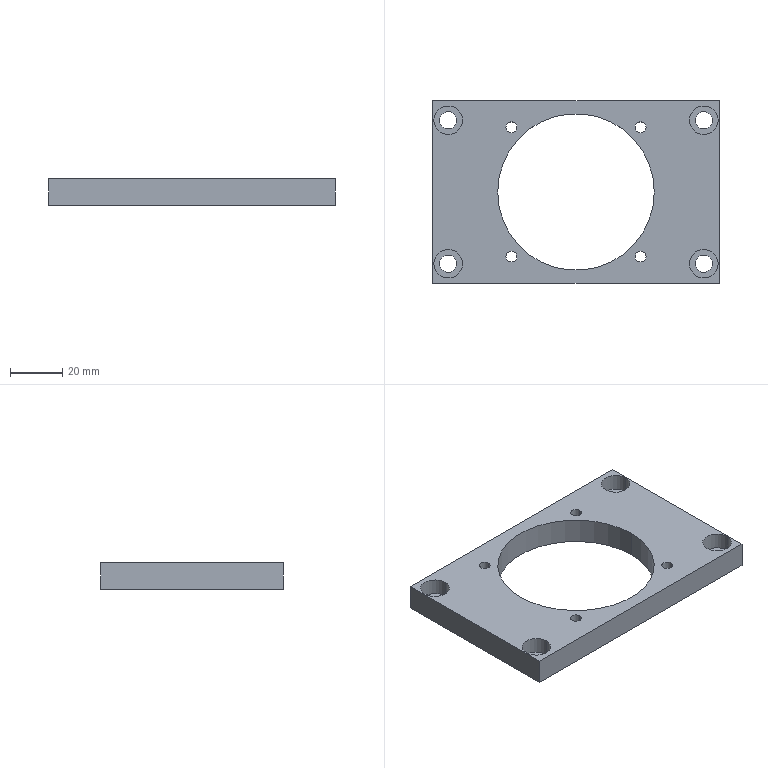Component | SolidWorks | ServoDriveMotorModule-1_WT-FLD-EJG-1212-00-019-1 | 1 solid | 36 faces | box 110 x 70 x 10 mm | volume 45246 mm3 | cylinder 26 | plane 10 | commonest cylinder face diameters 11 x8 6.6 x8 4.2 x8 60 x2 | material AISI 1045 Steel, cold drawn
STEP:
#1=COLOUR_RGB('',0.7922,0.8196,0.9333);
#2=FILL_AREA_STYLE_COLOUR('',#1);
#3=FILL_AREA_STYLE('',(#2));
#4=SURFACE_STYLE_FILL_AREA(#3);
#5=SURFACE_SIDE_STYLE('',(#4));
#6=SURFACE_STYLE_USAGE(.BOTH.,#5);
#7=PRESENTATION_STYLE_ASSIGNMENT((#6));
#8=CARTESIAN_POINT('',(-2.146,1.083,5.26));
#9=VERTEX_POINT('',#8);
#10=CARTESIAN_POINT('',(-1.713,1.083,5.26));
#11=VERTEX_POINT('',#10);
#12=CARTESIAN_POINT('',(-1.929,1.083,5.26));
#13=DIRECTION('',(0.,0.,1.));
#14=DIRECTION('',(1.,0.,0.));
#15=AXIS2_PLACEMENT_3D('',#12,#13,#14);
#16=CIRCLE('',#15,0.2165);
#17=EDGE_CURVE('',#9,#11,#16,.T.);
#18=ORIENTED_EDGE('',*,*,#17,.F.);
#19=CARTESIAN_POINT('',(-2.146,1.083,5.512));
#20=VERTEX_POINT('',#19);
#21=CARTESIAN_POINT('',(-2.146,1.083,5.512));
#22=DIRECTION('',(0.,0.,1.));
#23=VECTOR('',#22,39.37);
#24=LINE('',#21,#23);
#25=EDGE_CURVE('',#9,#20,#24,.T.);
#26=ORIENTED_EDGE('',*,*,#25,.T.);
#27=CARTESIAN_POINT('',(-1.713,1.083,5.512));
#28=VERTEX_POINT('',#27);
#29=CARTESIAN_POINT('',(-1.929,1.083,5.512));
#30=DIRECTION('',(0.,0.,1.));
#31=DIRECTION('',(1.,0.,0.));
#32=AXIS2_PLACEMENT_3D('',#29,#30,#31);
#33=CIRCLE('',#32,0.2165);
#34=EDGE_CURVE('',#20,#28,#33,.T.);
#35=ORIENTED_EDGE('',*,*,#34,.T.);
#36=CARTESIAN_POINT('',(-1.713,1.083,5.512));
#37=DIRECTION('',(0.,0.,1.));
#38=VECTOR('',#37,39.37);
#39=LINE('',#36,#38);
#40=EDGE_CURVE('',#11,#28,#39,.T.);
#41=ORIENTED_EDGE('',*,*,#40,.F.);
#42=EDGE_LOOP('',(#18,#26,#35,#41));
#43=FACE_OUTER_BOUND('',#42,.T.);
#44=CARTESIAN_POINT('',(-1.929,1.083,5.512));
#45=DIRECTION('',(0.,0.,1.));
#46=DIRECTION('',(1.,0.,0.));
#47=AXIS2_PLACEMENT_3D('',#44,#45,#46);
#48=CYLINDRICAL_SURFACE('',#47,0.2165);
#49=ADVANCED_FACE('',(#43),#48,.F.);
#50=CARTESIAN_POINT('',(-2.059,1.083,5.118));
#51=VERTEX_POINT('',#50);
#52=CARTESIAN_POINT('',(-1.799,1.083,5.118));
#53=VERTEX_POINT('',#52);
#54=CARTESIAN_POINT('',(-1.929,1.083,5.118));
#55=DIRECTION('',(0.,0.,1.));
#56=DIRECTION('',(1.,0.,0.));
#57=AXIS2_PLACEMENT_3D('',#54,#55,#56);
#58=CIRCLE('',#57,0.1299);
#59=EDGE_CURVE('',#51,#53,#58,.T.);
#60=ORIENTED_EDGE('',*,*,#59,.F.);
#61=CARTESIAN_POINT('',(-2.059,1.083,5.26));
#62=VERTEX_POINT('',#61);
#63=CARTESIAN_POINT('',(-2.059,1.083,5.512));
#64=DIRECTION('',(0.,0.,1.));
#65=VECTOR('',#64,39.37);
#66=LINE('',#63,#65);
#67=EDGE_CURVE('',#51,#62,#66,.T.);
#68=ORIENTED_EDGE('',*,*,#67,.T.);
#69=CARTESIAN_POINT('',(-1.799,1.083,5.26));
#70=VERTEX_POINT('',#69);
#71=CARTESIAN_POINT('',(-1.929,1.083,5.26));
#72=DIRECTION('',(0.,0.,1.));
#73=DIRECTION('',(1.,0.,0.));
#74=AXIS2_PLACEMENT_3D('',#71,#72,#73);
#75=CIRCLE('',#74,0.1299);
#76=EDGE_CURVE('',#62,#70,#75,.T.);
#77=ORIENTED_EDGE('',*,*,#76,.T.);
#78=CARTESIAN_POINT('',(-1.799,1.083,5.512));
#79=DIRECTION('',(0.,0.,1.));
#80=VECTOR('',#79,39.37);
#81=LINE('',#78,#80);
#82=EDGE_CURVE('',#53,#70,#81,.T.);
#83=ORIENTED_EDGE('',*,*,#82,.F.);
#84=EDGE_LOOP('',(#60,#68,#77,#83));
#85=FACE_OUTER_BOUND('',#84,.T.);
#86=CARTESIAN_POINT('',(-1.929,1.083,5.512));
#87=DIRECTION('',(0.,0.,1.));
#88=DIRECTION('',(1.,0.,0.));
#89=AXIS2_PLACEMENT_3D('',#86,#87,#88);
#90=CYLINDRICAL_SURFACE('',#89,0.1299);
#91=ADVANCED_FACE('',(#85),#90,.F.);
#92=CARTESIAN_POINT('',(-2.146,-1.083,5.26));
#93=VERTEX_POINT('',#92);
#94=CARTESIAN_POINT('',(-1.713,-1.083,5.26));
#95=VERTEX_POINT('',#94);
#96=CARTESIAN_POINT('',(-1.929,-1.083,5.26));
#97=DIRECTION('',(0.,0.,1.));
#98=DIRECTION('',(1.,0.,0.));
#99=AXIS2_PLACEMENT_3D('',#96,#97,#98);
#100=CIRCLE('',#99,0.2165);
#101=EDGE_CURVE('',#93,#95,#100,.T.);
#102=ORIENTED_EDGE('',*,*,#101,.F.);
#103=CARTESIAN_POINT('',(-2.146,-1.083,5.512));
#104=VERTEX_POINT('',#103);
#105=CARTESIAN_POINT('',(-2.146,-1.083,5.512));
#106=DIRECTION('',(0.,0.,1.));
#107=VECTOR('',#106,39.37);
#108=LINE('',#105,#107);
#109=EDGE_CURVE('',#93,#104,#108,.T.);
#110=ORIENTED_EDGE('',*,*,#109,.T.);
#111=CARTESIAN_POINT('',(-1.713,-1.083,5.512));
#112=VERTEX_POINT('',#111);
#113=CARTESIAN_POINT('',(-1.929,-1.083,5.512));
#114=DIRECTION('',(0.,0.,1.));
#115=DIRECTION('',(1.,0.,0.));
#116=AXIS2_PLACEMENT_3D('',#113,#114,#115);
#117=CIRCLE('',#116,0.2165);
#118=EDGE_CURVE('',#104,#112,#117,.T.);
#119=ORIENTED_EDGE('',*,*,#118,.T.);
#120=CARTESIAN_POINT('',(-1.713,-1.083,5.512));
#121=DIRECTION('',(0.,0.,1.));
#122=VECTOR('',#121,39.37);
#123=LINE('',#120,#122);
#124=EDGE_CURVE('',#95,#112,#123,.T.);
#125=ORIENTED_EDGE('',*,*,#124,.F.);
#126=EDGE_LOOP('',(#102,#110,#119,#125));
#127=FACE_OUTER_BOUND('',#126,.T.);
#128=CARTESIAN_POINT('',(-1.929,-1.083,5.512));
#129=DIRECTION('',(0.,0.,1.));
#130=DIRECTION('',(1.,0.,0.));
#131=AXIS2_PLACEMENT_3D('',#128,#129,#130);
#132=CYLINDRICAL_SURFACE('',#131,0.2165);
#133=ADVANCED_FACE('',(#127),#132,.F.);
#134=CARTESIAN_POINT('',(-2.059,-1.083,5.118));
#135=VERTEX_POINT('',#134);
#136=CARTESIAN_POINT('',(-1.799,-1.083,5.118));
#137=VERTEX_POINT('',#136);
#138=CARTESIAN_POINT('',(-1.929,-1.083,5.118));
#139=DIRECTION('',(0.,0.,1.));
#140=DIRECTION('',(1.,0.,0.));
#141=AXIS2_PLACEMENT_3D('',#138,#139,#140);
#142=CIRCLE('',#141,0.1299);
#143=EDGE_CURVE('',#135,#137,#142,.T.);
#144=ORIENTED_EDGE('',*,*,#143,.F.);
#145=CARTESIAN_POINT('',(-2.059,-1.083,5.26));
#146=VERTEX_POINT('',#145);
#147=CARTESIAN_POINT('',(-2.059,-1.083,5.512));
#148=DIRECTION('',(0.,0.,1.));
#149=VECTOR('',#148,39.37);
#150=LINE('',#147,#149);
#151=EDGE_CURVE('',#135,#146,#150,.T.);
#152=ORIENTED_EDGE('',*,*,#151,.T.);
#153=CARTESIAN_POINT('',(-1.799,-1.083,5.26));
#154=VERTEX_POINT('',#153);
#155=CARTESIAN_POINT('',(-1.929,-1.083,5.26));
#156=DIRECTION('',(0.,0.,1.));
#157=DIRECTION('',(1.,0.,0.));
#158=AXIS2_PLACEMENT_3D('',#155,#156,#157);
#159=CIRCLE('',#158,0.1299);
#160=EDGE_CURVE('',#146,#154,#159,.T.);
#161=ORIENTED_EDGE('',*,*,#160,.T.);
#162=CARTESIAN_POINT('',(-1.799,-1.083,5.512));
#163=DIRECTION('',(0.,0.,1.));
#164=VECTOR('',#163,39.37);
#165=LINE('',#162,#164);
#166=EDGE_CURVE('',#137,#154,#165,.T.);
#167=ORIENTED_EDGE('',*,*,#166,.F.);
#168=EDGE_LOOP('',(#144,#152,#161,#167));
#169=FACE_OUTER_BOUND('',#168,.T.);
#170=CARTESIAN_POINT('',(-1.929,-1.083,5.512));
#171=DIRECTION('',(0.,0.,1.));
#172=DIRECTION('',(1.,0.,0.));
#173=AXIS2_PLACEMENT_3D('',#170,#171,#172);
#174=CYLINDRICAL_SURFACE('',#173,0.1299);
#175=ADVANCED_FACE('',(#169),#174,.F.);
#176=CARTESIAN_POINT('',(1.713,-1.083,5.26));
#177=VERTEX_POINT('',#176);
#178=CARTESIAN_POINT('',(2.146,-1.083,5.26));
#179=VERTEX_POINT('',#178);
#180=CARTESIAN_POINT('',(1.929,-1.083,5.26));
#181=DIRECTION('',(0.,0.,1.));
#182=DIRECTION('',(1.,0.,0.));
#183=AXIS2_PLACEMENT_3D('',#180,#181,#182);
#184=CIRCLE('',#183,0.2165);
#185=EDGE_CURVE('',#177,#179,#184,.T.);
#186=ORIENTED_EDGE('',*,*,#185,.F.);
#187=CARTESIAN_POINT('',(1.713,-1.083,5.512));
#188=VERTEX_POINT('',#187);
#189=CARTESIAN_POINT('',(1.713,-1.083,5.512));
#190=DIRECTION('',(0.,0.,1.));
#191=VECTOR('',#190,39.37);
#192=LINE('',#189,#191);
#193=EDGE_CURVE('',#177,#188,#192,.T.);
#194=ORIENTED_EDGE('',*,*,#193,.T.);
#195=CARTESIAN_POINT('',(2.146,-1.083,5.512));
#196=VERTEX_POINT('',#195);
#197=CARTESIAN_POINT('',(1.929,-1.083,5.512));
#198=DIRECTION('',(0.,0.,1.));
#199=DIRECTION('',(1.,0.,0.));
#200=AXIS2_PLACEMENT_3D('',#197,#198,#199);
#201=CIRCLE('',#200,0.2165);
#202=EDGE_CURVE('',#188,#196,#201,.T.);
#203=ORIENTED_EDGE('',*,*,#202,.T.);
#204=CARTESIAN_POINT('',(2.146,-1.083,5.512));
#205=DIRECTION('',(0.,0.,1.));
#206=VECTOR('',#205,39.37);
#207=LINE('',#204,#206);
#208=EDGE_CURVE('',#179,#196,#207,.T.);
#209=ORIENTED_EDGE('',*,*,#208,.F.);
#210=EDGE_LOOP('',(#186,#194,#203,#209));
#211=FACE_OUTER_BOUND('',#210,.T.);
#212=CARTESIAN_POINT('',(1.929,-1.083,5.512));
#213=DIRECTION('',(0.,0.,1.));
#214=DIRECTION('',(1.,0.,0.));
#215=AXIS2_PLACEMENT_3D('',#212,#213,#214);
#216=CYLINDRICAL_SURFACE('',#215,0.2165);
#217=ADVANCED_FACE('',(#211),#216,.F.);
#218=CARTESIAN_POINT('',(1.799,-1.083,5.118));
#219=VERTEX_POINT('',#218);
#220=CARTESIAN_POINT('',(2.059,-1.083,5.118));
#221=VERTEX_POINT('',#220);
#222=CARTESIAN_POINT('',(1.929,-1.083,5.118));
#223=DIRECTION('',(0.,0.,1.));
#224=DIRECTION('',(1.,0.,0.));
#225=AXIS2_PLACEMENT_3D('',#222,#223,#224);
#226=CIRCLE('',#225,0.1299);
#227=EDGE_CURVE('',#219,#221,#226,.T.);
#228=ORIENTED_EDGE('',*,*,#227,.F.);
#229=CARTESIAN_POINT('',(1.799,-1.083,5.26));
#230=VERTEX_POINT('',#229);
#231=CARTESIAN_POINT('',(1.799,-1.083,5.512));
#232=DIRECTION('',(0.,0.,1.));
#233=VECTOR('',#232,39.37);
#234=LINE('',#231,#233);
#235=EDGE_CURVE('',#219,#230,#234,.T.);
#236=ORIENTED_EDGE('',*,*,#235,.T.);
#237=CARTESIAN_POINT('',(2.059,-1.083,5.26));
#238=VERTEX_POINT('',#237);
#239=CARTESIAN_POINT('',(1.929,-1.083,5.26));
#240=DIRECTION('',(0.,0.,1.));
#241=DIRECTION('',(1.,0.,0.));
#242=AXIS2_PLACEMENT_3D('',#239,#240,#241);
#243=CIRCLE('',#242,0.1299);
#244=EDGE_CURVE('',#230,#238,#243,.T.);
#245=ORIENTED_EDGE('',*,*,#244,.T.);
#246=CARTESIAN_POINT('',(2.059,-1.083,5.512));
#247=DIRECTION('',(0.,0.,1.));
#248=VECTOR('',#247,39.37);
#249=LINE('',#246,#248);
#250=EDGE_CURVE('',#221,#238,#249,.T.);
#251=ORIENTED_EDGE('',*,*,#250,.F.);
#252=EDGE_LOOP('',(#228,#236,#245,#251));
#253=FACE_OUTER_BOUND('',#252,.T.);
#254=CARTESIAN_POINT('',(1.929,-1.083,5.512));
#255=DIRECTION('',(0.,0.,1.));
#256=DIRECTION('',(1.,0.,0.));
#257=AXIS2_PLACEMENT_3D('',#254,#255,#256);
#258=CYLINDRICAL_SURFACE('',#257,0.1299);
#259=ADVANCED_FACE('',(#253),#258,.F.);
#260=CARTESIAN_POINT('',(1.713,1.083,5.26));
#261=VERTEX_POINT('',#260);
#262=CARTESIAN_POINT('',(2.146,1.083,5.26));
#263=VERTEX_POINT('',#262);
#264=CARTESIAN_POINT('',(1.929,1.083,5.26));
#265=DIRECTION('',(0.,0.,1.));
#266=DIRECTION('',(1.,0.,0.));
#267=AXIS2_PLACEMENT_3D('',#264,#265,#266);
#268=CIRCLE('',#267,0.2165);
#269=EDGE_CURVE('',#261,#263,#268,.T.);
#270=ORIENTED_EDGE('',*,*,#269,.F.);
#271=CARTESIAN_POINT('',(1.713,1.083,5.512));
#272=VERTEX_POINT('',#271);
#273=CARTESIAN_POINT('',(1.713,1.083,5.512));
#274=DIRECTION('',(0.,0.,1.));
#275=VECTOR('',#274,39.37);
#276=LINE('',#273,#275);
#277=EDGE_CURVE('',#261,#272,#276,.T.);
#278=ORIENTED_EDGE('',*,*,#277,.T.);
#279=CARTESIAN_POINT('',(2.146,1.083,5.512));
#280=VERTEX_POINT('',#279);
#281=CARTESIAN_POINT('',(1.929,1.083,5.512));
#282=DIRECTION('',(0.,0.,1.));
#283=DIRECTION('',(1.,0.,0.));
#284=AXIS2_PLACEMENT_3D('',#281,#282,#283);
#285=CIRCLE('',#284,0.2165);
#286=EDGE_CURVE('',#272,#280,#285,.T.);
#287=ORIENTED_EDGE('',*,*,#286,.T.);
#288=CARTESIAN_POINT('',(2.146,1.083,5.512));
#289=DIRECTION('',(0.,0.,1.));
#290=VECTOR('',#289,39.37);
#291=LINE('',#288,#290);
#292=EDGE_CURVE('',#263,#280,#291,.T.);
#293=ORIENTED_EDGE('',*,*,#292,.F.);
#294=EDGE_LOOP('',(#270,#278,#287,#293));
#295=FACE_OUTER_BOUND('',#294,.T.);
#296=CARTESIAN_POINT('',(1.929,1.083,5.512));
#297=DIRECTION('',(0.,0.,1.));
#298=DIRECTION('',(1.,0.,0.));
#299=AXIS2_PLACEMENT_3D('',#296,#297,#298);
#300=CYLINDRICAL_SURFACE('',#299,0.2165);
#301=ADVANCED_FACE('',(#295),#300,.F.);
#302=CARTESIAN_POINT('',(1.799,1.083,5.118));
#303=VERTEX_POINT('',#302);
#304=CARTESIAN_POINT('',(2.059,1.083,5.118));
#305=VERTEX_POINT('',#304);
#306=CARTESIAN_POINT('',(1.929,1.083,5.118));
#307=DIRECTION('',(0.,0.,1.));
#308=DIRECTION('',(1.,0.,0.));
#309=AXIS2_PLACEMENT_3D('',#306,#307,#308);
#310=CIRCLE('',#309,0.1299);
#311=EDGE_CURVE('',#303,#305,#310,.T.);
#312=ORIENTED_EDGE('',*,*,#311,.F.);
#313=CARTESIAN_POINT('',(1.799,1.083,5.26));
#314=VERTEX_POINT('',#313);
#315=CARTESIAN_POINT('',(1.799,1.083,5.512));
#316=DIRECTION('',(0.,0.,1.));
#317=VECTOR('',#316,39.37);
#318=LINE('',#315,#317);
#319=EDGE_CURVE('',#303,#314,#318,.T.);
#320=ORIENTED_EDGE('',*,*,#319,.T.);
#321=CARTESIAN_POINT('',(2.059,1.083,5.26));
#322=VERTEX_POINT('',#321);
#323=CARTESIAN_POINT('',(1.929,1.083,5.26));
#324=DIRECTION('',(0.,0.,1.));
#325=DIRECTION('',(1.,0.,0.));
#326=AXIS2_PLACEMENT_3D('',#323,#324,#325);
#327=CIRCLE('',#326,0.1299);
#328=EDGE_CURVE('',#314,#322,#327,.T.);
#329=ORIENTED_EDGE('',*,*,#328,.T.);
#330=CARTESIAN_POINT('',(2.059,1.083,5.512));
#331=DIRECTION('',(0.,0.,1.));
#332=VECTOR('',#331,39.37);
#333=LINE('',#330,#332);
#334=EDGE_CURVE('',#305,#322,#333,.T.);
#335=ORIENTED_EDGE('',*,*,#334,.F.);
#336=EDGE_LOOP('',(#312,#320,#329,#335));
#337=FACE_OUTER_BOUND('',#336,.T.);
#338=CARTESIAN_POINT('',(1.929,1.083,5.512));
#339=DIRECTION('',(0.,0.,1.));
#340=DIRECTION('',(1.,0.,0.));
#341=AXIS2_PLACEMENT_3D('',#338,#339,#340);
#342=CYLINDRICAL_SURFACE('',#341,0.1299);
#343=ADVANCED_FACE('',(#337),#342,.F.);
#344=CARTESIAN_POINT('',(0.8917,-0.9744,5.118));
#345=VERTEX_POINT('',#344);
#346=CARTESIAN_POINT('',(1.057,-0.9744,5.118));
#347=VERTEX_POINT('',#346);
#348=CARTESIAN_POINT('',(0.9744,-0.9744,5.118));
#349=DIRECTION('',(0.,0.,1.));
#350=DIRECTION('',(1.,0.,0.));
#351=AXIS2_PLACEMENT_3D('',#348,#349,#350);
#352=CIRCLE('',#351,0.08268);
#353=EDGE_CURVE('',#345,#347,#352,.T.);
#354=ORIENTED_EDGE('',*,*,#353,.F.);
#355=CARTESIAN_POINT('',(0.8917,-0.9744,5.512));
#356=VERTEX_POINT('',#355);
#357=CARTESIAN_POINT('',(0.8917,-0.9744,5.512));
#358=DIRECTION('',(0.,0.,1.));
#359=VECTOR('',#358,39.37);
#360=LINE('',#357,#359);
#361=EDGE_CURVE('',#345,#356,#360,.T.);
#362=ORIENTED_EDGE('',*,*,#361,.T.);
#363=CARTESIAN_POINT('',(1.057,-0.9744,5.512));
#364=VERTEX_POINT('',#363);
#365=CARTESIAN_POINT('',(0.9744,-0.9744,5.512));
#366=DIRECTION('',(0.,0.,1.));
#367=DIRECTION('',(1.,0.,0.));
#368=AXIS2_PLACEMENT_3D('',#365,#366,#367);
#369=CIRCLE('',#368,0.08268);
#370=EDGE_CURVE('',#356,#364,#369,.T.);
#371=ORIENTED_EDGE('',*,*,#370,.T.);
#372=CARTESIAN_POINT('',(1.057,-0.9744,5.512));
#373=DIRECTION('',(0.,0.,1.));
#374=VECTOR('',#373,39.37);
#375=LINE('',#372,#374);
#376=EDGE_CURVE('',#347,#364,#375,.T.);
#377=ORIENTED_EDGE('',*,*,#376,.F.);
#378=EDGE_LOOP('',(#354,#362,#371,#377));
#379=FACE_OUTER_BOUND('',#378,.T.);
#380=CARTESIAN_POINT('',(0.9744,-0.9744,5.512));
#381=DIRECTION('',(0.,0.,1.));
#382=DIRECTION('',(1.,0.,0.));
#383=AXIS2_PLACEMENT_3D('',#380,#381,#382);
#384=CYLINDRICAL_SURFACE('',#383,0.08268);
#385=ADVANCED_FACE('',(#379),#384,.F.);
#386=CARTESIAN_POINT('',(-1.057,0.9744,5.118));
#387=VERTEX_POINT('',#386);
#388=CARTESIAN_POINT('',(-0.8917,0.9744,5.118));
#389=VERTEX_POINT('',#388);
#390=CARTESIAN_POINT('',(-0.9744,0.9744,5.118));
#391=DIRECTION('',(0.,0.,1.));
#392=DIRECTION('',(1.,0.,0.));
#393=AXIS2_PLACEMENT_3D('',#390,#391,#392);
#394=CIRCLE('',#393,0.08268);
#395=EDGE_CURVE('',#387,#389,#394,.T.);
#396=ORIENTED_EDGE('',*,*,#395,.F.);
#397=CARTESIAN_POINT('',(-1.057,0.9744,5.512));
#398=VERTEX_POINT('',#397);
#399=CARTESIAN_POINT('',(-1.057,0.9744,5.512));
#400=DIRECTION('',(0.,0.,1.));
#401=VECTOR('',#400,39.37);
#402=LINE('',#399,#401);
#403=EDGE_CURVE('',#387,#398,#402,.T.);
#404=ORIENTED_EDGE('',*,*,#403,.T.);
#405=CARTESIAN_POINT('',(-0.8917,0.9744,5.512));
#406=VERTEX_POINT('',#405);
#407=CARTESIAN_POINT('',(-0.9744,0.9744,5.512));
#408=DIRECTION('',(0.,0.,1.));
#409=DIRECTION('',(1.,0.,0.));
#410=AXIS2_PLACEMENT_3D('',#407,#408,#409);
#411=CIRCLE('',#410,0.08268);
#412=EDGE_CURVE('',#398,#406,#411,.T.);
#413=ORIENTED_EDGE('',*,*,#412,.T.);
#414=CARTESIAN_POINT('',(-0.8917,0.9744,5.512));
#415=DIRECTION('',(0.,0.,1.));
#416=VECTOR('',#415,39.37);
#417=LINE('',#414,#416);
#418=EDGE_CURVE('',#389,#406,#417,.T.);
#419=ORIENTED_EDGE('',*,*,#418,.F.);
#420=EDGE_LOOP('',(#396,#404,#413,#419));
#421=FACE_OUTER_BOUND('',#420,.T.);
#422=CARTESIAN_POINT('',(-0.9744,0.9744,5.512));
#423=DIRECTION('',(0.,0.,1.));
#424=DIRECTION('',(1.,0.,0.));
#425=AXIS2_PLACEMENT_3D('',#422,#423,#424);
#426=CYLINDRICAL_SURFACE('',#425,0.08268);
#427=ADVANCED_FACE('',(#421),#426,.F.);
#428=CARTESIAN_POINT('',(-1.057,-0.9744,5.118));
#429=VERTEX_POINT('',#428);
#430=CARTESIAN_POINT('',(-0.8917,-0.9744,5.118));
#431=VERTEX_POINT('',#430);
#432=CARTESIAN_POINT('',(-0.9744,-0.9744,5.118));
#433=DIRECTION('',(0.,0.,1.));
#434=DIRECTION('',(1.,0.,0.));
#435=AXIS2_PLACEMENT_3D('',#432,#433,#434);
#436=CIRCLE('',#435,0.08268);
#437=EDGE_CURVE('',#429,#431,#436,.T.);
#438=ORIENTED_EDGE('',*,*,#437,.F.);
#439=CARTESIAN_POINT('',(-1.057,-0.9744,5.512));
#440=VERTEX_POINT('',#439);
#441=CARTESIAN_POINT('',(-1.057,-0.9744,5.512));
#442=DIRECTION('',(0.,0.,1.));
#443=VECTOR('',#442,39.37);
#444=LINE('',#441,#443);
#445=EDGE_CURVE('',#429,#440,#444,.T.);
#446=ORIENTED_EDGE('',*,*,#445,.T.);
#447=CARTESIAN_POINT('',(-0.8917,-0.9744,5.512));
#448=VERTEX_POINT('',#447);
#449=CARTESIAN_POINT('',(-0.9744,-0.9744,5.512));
#450=DIRECTION('',(0.,0.,1.));
#451=DIRECTION('',(1.,0.,0.));
#452=AXIS2_PLACEMENT_3D('',#449,#450,#451);
#453=CIRCLE('',#452,0.08268);
#454=EDGE_CURVE('',#440,#448,#453,.T.);
#455=ORIENTED_EDGE('',*,*,#454,.T.);
#456=CARTESIAN_POINT('',(-0.8917,-0.9744,5.512));
#457=DIRECTION('',(0.,0.,1.));
#458=VECTOR('',#457,39.37);
#459=LINE('',#456,#458);
#460=EDGE_CURVE('',#431,#448,#459,.T.);
#461=ORIENTED_EDGE('',*,*,#460,.F.);
#462=EDGE_LOOP('',(#438,#446,#455,#461));
#463=FACE_OUTER_BOUND('',#462,.T.);
#464=CARTESIAN_POINT('',(-0.9744,-0.9744,5.512));
#465=DIRECTION('',(0.,0.,1.));
#466=DIRECTION('',(1.,0.,0.));
#467=AXIS2_PLACEMENT_3D('',#464,#465,#466);
#468=CYLINDRICAL_SURFACE('',#467,0.08268);
#469=ADVANCED_FACE('',(#463),#468,.F.);
#470=CARTESIAN_POINT('',(0.8917,0.9744,5.118));
#471=VERTEX_POINT('',#470);
#472=CARTESIAN_POINT('',(1.057,0.9744,5.118));
#473=VERTEX_POINT('',#472);
#474=CARTESIAN_POINT('',(0.9744,0.9744,5.118));
#475=DIRECTION('',(0.,0.,1.));
#476=DIRECTION('',(1.,0.,0.));
#477=AXIS2_PLACEMENT_3D('',#474,#475,#476);
#478=CIRCLE('',#477,0.08268);
#479=EDGE_CURVE('',#471,#473,#478,.T.);
#480=ORIENTED_EDGE('',*,*,#479,.F.);
#481=CARTESIAN_POINT('',(0.8917,0.9744,5.512));
#482=VERTEX_POINT('',#481);
#483=CARTESIAN_POINT('',(0.8917,0.9744,5.512));
#484=DIRECTION('',(0.,0.,1.));
#485=VECTOR('',#484,39.37);
#486=LINE('',#483,#485);
#487=EDGE_CURVE('',#471,#482,#486,.T.);
#488=ORIENTED_EDGE('',*,*,#487,.T.);
#489=CARTESIAN_POINT('',(1.057,0.9744,5.512));
#490=VERTEX_POINT('',#489);
#491=CARTESIAN_POINT('',(0.9744,0.9744,5.512));
#492=DIRECTION('',(0.,0.,1.));
#493=DIRECTION('',(1.,0.,0.));
#494=AXIS2_PLACEMENT_3D('',#491,#492,#493);
#495=CIRCLE('',#494,0.08268);
#496=EDGE_CURVE('',#482,#490,#495,.T.);
#497=ORIENTED_EDGE('',*,*,#496,.T.);
#498=CARTESIAN_POINT('',(1.057,0.9744,5.512));
#499=DIRECTION('',(0.,0.,1.));
#500=VECTOR('',#499,39.37);
#501=LINE('',#498,#500);
#502=EDGE_CURVE('',#473,#490,#501,.T.);
#503=ORIENTED_EDGE('',*,*,#502,.F.);
#504=EDGE_LOOP('',(#480,#488,#497,#503));
#505=FACE_OUTER_BOUND('',#504,.T.);
#506=CARTESIAN_POINT('',(0.9744,0.9744,5.512));
#507=DIRECTION('',(0.,0.,1.));
#508=DIRECTION('',(1.,0.,0.));
#509=AXIS2_PLACEMENT_3D('',#506,#507,#508);
#510=CYLINDRICAL_SURFACE('',#509,0.08268);
#511=ADVANCED_FACE('',(#505),#510,.F.);
#512=CARTESIAN_POINT('',(-1.181,-0.,5.118));
#513=VERTEX_POINT('',#512);
#514=CARTESIAN_POINT('',(1.181,-0.,5.118));
#515=VERTEX_POINT('',#514);
#516=CARTESIAN_POINT('',(0.,-0.,5.118));
#517=DIRECTION('',(0.,0.,1.));
#518=DIRECTION('',(1.,0.,0.));
#519=AXIS2_PLACEMENT_3D('',#516,#517,#518);
#520=CIRCLE('',#519,1.181);
#521=EDGE_CURVE('',#513,#515,#520,.T.);
#522=ORIENTED_EDGE('',*,*,#521,.F.);
#523=CARTESIAN_POINT('',(-1.181,-0.,5.512));
#524=VERTEX_POINT('',#523);
#525=CARTESIAN_POINT('',(-1.181,-0.,5.118));
#526=DIRECTION('',(0.,0.,1.));
#527=VECTOR('',#526,39.37);
#528=LINE('',#525,#527);
#529=EDGE_CURVE('',#513,#524,#528,.T.);
#530=ORIENTED_EDGE('',*,*,#529,.T.);
#531=CARTESIAN_POINT('',(1.181,-0.,5.512));
#532=VERTEX_POINT('',#531);
#533=CARTESIAN_POINT('',(0.,-0.,5.512));
#534=DIRECTION('',(0.,0.,1.));
#535=DIRECTION('',(1.,0.,0.));
#536=AXIS2_PLACEMENT_3D('',#533,#534,#535);
#537=CIRCLE('',#536,1.181);
#538=EDGE_CURVE('',#524,#532,#537,.T.);
#539=ORIENTED_EDGE('',*,*,#538,.T.);
#540=CARTESIAN_POINT('',(1.181,-0.,5.118));
#541=DIRECTION('',(0.,0.,1.));
#542=VECTOR('',#541,39.37);
#543=LINE('',#540,#542);
#544=EDGE_CURVE('',#515,#532,#543,.T.);
#545=ORIENTED_EDGE('',*,*,#544,.F.);
#546=EDGE_LOOP('',(#522,#530,#539,#545));
#547=FACE_OUTER_BOUND('',#546,.T.);
#548=CARTESIAN_POINT('',(0.,-0.,5.118));
#549=DIRECTION('',(0.,0.,1.));
#550=DIRECTION('',(1.,0.,0.));
#551=AXIS2_PLACEMENT_3D('',#548,#549,#550);
#552=CYLINDRICAL_SURFACE('',#551,1.181);
#553=ADVANCED_FACE('',(#547),#552,.F.);
#554=CARTESIAN_POINT('',(2.165,-1.378,5.118));
#555=VERTEX_POINT('',#554);
#556=CARTESIAN_POINT('',(2.165,1.378,5.118));
#557=VERTEX_POINT('',#556);
#558=CARTESIAN_POINT('',(2.165,1.378,5.118));
#559=DIRECTION('',(-0.,1.,0.));
#560=VECTOR('',#559,39.37);
#561=LINE('',#558,#560);
#562=EDGE_CURVE('',#555,#557,#561,.T.);
#563=ORIENTED_EDGE('',*,*,#562,.T.);
#564=CARTESIAN_POINT('',(2.165,1.378,5.512));
#565=VERTEX_POINT('',#564);
#566=CARTESIAN_POINT('',(2.165,1.378,5.512));
#567=DIRECTION('',(0.,0.,-1.));
#568=VECTOR('',#567,39.37);
#569=LINE('',#566,#568);
#570=EDGE_CURVE('',#565,#557,#569,.T.);
#571=ORIENTED_EDGE('',*,*,#570,.F.);
#572=CARTESIAN_POINT('',(2.165,-1.378,5.512));
#573=VERTEX_POINT('',#572);
#574=CARTESIAN_POINT('',(2.165,1.378,5.512));
#575=DIRECTION('',(-0.,1.,0.));
#576=VECTOR('',#575,39.37);
#577=LINE('',#574,#576);
#578=EDGE_CURVE('',#573,#565,#577,.T.);
#579=ORIENTED_EDGE('',*,*,#578,.F.);
#580=CARTESIAN_POINT('',(2.165,-1.378,5.512));
#581=DIRECTION('',(0.,0.,-1.));
#582=VECTOR('',#581,39.37);
#583=LINE('',#580,#582);
#584=EDGE_CURVE('',#573,#555,#583,.T.);
#585=ORIENTED_EDGE('',*,*,#584,.T.);
#586=EDGE_LOOP('',(#563,#571,#579,#585));
#587=FACE_OUTER_BOUND('',#586,.T.);
#588=CARTESIAN_POINT('',(2.165,1.378,5.512));
#589=DIRECTION('',(-1.,-0.,0.));
#590=DIRECTION('',(0.,-1.,0.));
#591=AXIS2_PLACEMENT_3D('',#588,#589,#590);
#592=PLANE('',#591);
#593=ADVANCED_FACE('',(#587),#592,.F.);
#594=CARTESIAN_POINT('',(-2.165,1.378,5.118));
#595=VERTEX_POINT('',#594);
#596=CARTESIAN_POINT('',(-2.165,1.378,5.118));
#597=DIRECTION('',(-1.,-0.,0.));
#598=VECTOR('',#597,39.37);
#599=LINE('',#596,#598);
#600=EDGE_CURVE('',#557,#595,#599,.T.);
#601=ORIENTED_EDGE('',*,*,#600,.T.);
#602=CARTESIAN_POINT('',(-2.165,1.378,5.512));
#603=VERTEX_POINT('',#602);
#604=CARTESIAN_POINT('',(-2.165,1.378,5.512));
#605=DIRECTION('',(0.,0.,-1.));
#606=VECTOR('',#605,39.37);
#607=LINE('',#604,#606);
#608=EDGE_CURVE('',#603,#595,#607,.T.);
#609=ORIENTED_EDGE('',*,*,#608,.F.);
#610=CARTESIAN_POINT('',(-2.165,1.378,5.512));
#611=DIRECTION('',(-1.,-0.,0.));
#612=VECTOR('',#611,39.37);
#613=LINE('',#610,#612);
#614=EDGE_CURVE('',#565,#603,#613,.T.);
#615=ORIENTED_EDGE('',*,*,#614,.F.);
#616=ORIENTED_EDGE('',*,*,#570,.T.);
#617=EDGE_LOOP('',(#601,#609,#615,#616));
#618=FACE_OUTER_BOUND('',#617,.T.);
#619=CARTESIAN_POINT('',(-2.165,1.378,5.512));
#620=DIRECTION('',(0.,-1.,0.));
#621=DIRECTION('',(1.,0.,0.));
#622=AXIS2_PLACEMENT_3D('',#619,#620,#621);
#623=PLANE('',#622);
#624=ADVANCED_FACE('',(#618),#623,.F.);
#625=CARTESIAN_POINT('',(-2.165,-1.378,5.118));
#626=VERTEX_POINT('',#625);
#627=CARTESIAN_POINT('',(-2.165,1.378,5.118));
#628=DIRECTION('',(0.,-1.,0.));
#629=VECTOR('',#628,39.37);
#630=LINE('',#627,#629);
#631=EDGE_CURVE('',#595,#626,#630,.T.);
#632=ORIENTED_EDGE('',*,*,#631,.T.);
#633=CARTESIAN_POINT('',(-2.165,-1.378,5.512));
#634=VERTEX_POINT('',#633);
#635=CARTESIAN_POINT('',(-2.165,-1.378,5.512));
#636=DIRECTION('',(0.,0.,-1.));
#637=VECTOR('',#636,39.37);
#638=LINE('',#635,#637);
#639=EDGE_CURVE('',#634,#626,#638,.T.);
#640=ORIENTED_EDGE('',*,*,#639,.F.);
#641=CARTESIAN_POINT('',(-2.165,1.378,5.512));
#642=DIRECTION('',(0.,-1.,0.));
#643=VECTOR('',#642,39.37);
#644=LINE('',#641,#643);
#645=EDGE_CURVE('',#603,#634,#644,.T.);
#646=ORIENTED_EDGE('',*,*,#645,.F.);
#647=ORIENTED_EDGE('',*,*,#608,.T.);
#648=EDGE_LOOP('',(#632,#640,#646,#647));
#649=FACE_OUTER_BOUND('',#648,.T.);
#650=CARTESIAN_POINT('',(-2.165,1.378,5.512));
#651=DIRECTION('',(1.,0.,0.));
#652=DIRECTION('',(-0.,1.,0.));
#653=AXIS2_PLACEMENT_3D('',#650,#651,#652);
#654=PLANE('',#653);
#655=ADVANCED_FACE('',(#649),#654,.F.);
#656=CARTESIAN_POINT('',(-2.165,-1.378,5.118));
#657=DIRECTION('',(1.,0.,0.));
#658=VECTOR('',#657,39.37);
#659=LINE('',#656,#658);
#660=EDGE_CURVE('',#626,#555,#659,.T.);
#661=ORIENTED_EDGE('',*,*,#660,.T.);
#662=ORIENTED_EDGE('',*,*,#584,.F.);
#663=CARTESIAN_POINT('',(-2.165,-1.378,5.512));
#664=DIRECTION('',(1.,0.,0.));
#665=VECTOR('',#664,39.37);
#666=LINE('',#663,#665);
#667=EDGE_CURVE('',#634,#573,#666,.T.);
#668=ORIENTED_EDGE('',*,*,#667,.F.);
#669=ORIENTED_EDGE('',*,*,#639,.T.);
#670=EDGE_LOOP('',(#661,#662,#668,#669));
#671=FACE_OUTER_BOUND('',#670,.T.);
#672=CARTESIAN_POINT('',(-2.165,-1.378,5.512));
#673=DIRECTION('',(0.,1.,0.));
#674=DIRECTION('',(0.,0.,1.));
#675=AXIS2_PLACEMENT_3D('',#672,#673,#674);
#676=PLANE('',#675);
#677=ADVANCED_FACE('',(#671),#676,.F.);
#678=CARTESIAN_POINT('',(-1.929,1.083,5.512));
#679=DIRECTION('',(0.,0.,1.));
#680=DIRECTION('',(1.,0.,0.));
#681=AXIS2_PLACEMENT_3D('',#678,#679,#680);
#682=CIRCLE('',#681,0.2165);
#683=EDGE_CURVE('',#28,#20,#682,.T.);
#684=ORIENTED_EDGE('',*,*,#683,.F.);
#685=ORIENTED_EDGE('',*,*,#34,.F.);
#686=EDGE_LOOP('',(#684,#685));
#687=FACE_BOUND('',#686,.T.);
#688=CARTESIAN_POINT('',(-1.929,-1.083,5.512));
#689=DIRECTION('',(0.,0.,1.));
#690=DIRECTION('',(1.,0.,0.));
#691=AXIS2_PLACEMENT_3D('',#688,#689,#690);
#692=CIRCLE('',#691,0.2165);
#693=EDGE_CURVE('',#112,#104,#692,.T.);
#694=ORIENTED_EDGE('',*,*,#693,.F.);
#695=ORIENTED_EDGE('',*,*,#118,.F.);
#696=EDGE_LOOP('',(#694,#695));
#697=FACE_BOUND('',#696,.T.);
#698=CARTESIAN_POINT('',(1.929,-1.083,5.512));
#699=DIRECTION('',(0.,0.,1.));
#700=DIRECTION('',(1.,0.,0.));
#701=AXIS2_PLACEMENT_3D('',#698,#699,#700);
#702=CIRCLE('',#701,0.2165);
#703=EDGE_CURVE('',#196,#188,#702,.T.);
#704=ORIENTED_EDGE('',*,*,#703,.F.);
#705=ORIENTED_EDGE('',*,*,#202,.F.);
#706=EDGE_LOOP('',(#704,#705));
#707=FACE_BOUND('',#706,.T.);
#708=CARTESIAN_POINT('',(1.929,1.083,5.512));
#709=DIRECTION('',(0.,0.,1.));
#710=DIRECTION('',(1.,0.,0.));
#711=AXIS2_PLACEMENT_3D('',#708,#709,#710);
#712=CIRCLE('',#711,0.2165);
#713=EDGE_CURVE('',#280,#272,#712,.T.);
#714=ORIENTED_EDGE('',*,*,#713,.F.);
#715=ORIENTED_EDGE('',*,*,#286,.F.);
#716=EDGE_LOOP('',(#714,#715));
#717=FACE_BOUND('',#716,.T.);
#718=CARTESIAN_POINT('',(0.9744,-0.9744,5.512));
#719=DIRECTION('',(0.,0.,1.));
#720=DIRECTION('',(1.,0.,0.));
#721=AXIS2_PLACEMENT_3D('',#718,#719,#720);
#722=CIRCLE('',#721,0.08268);
#723=EDGE_CURVE('',#364,#356,#722,.T.);
#724=ORIENTED_EDGE('',*,*,#723,.F.);
#725=ORIENTED_EDGE('',*,*,#370,.F.);
#726=EDGE_LOOP('',(#724,#725));
#727=FACE_BOUND('',#726,.T.);
#728=CARTESIAN_POINT('',(-0.9744,0.9744,5.512));
#729=DIRECTION('',(0.,0.,1.));
#730=DIRECTION('',(1.,0.,0.));
#731=AXIS2_PLACEMENT_3D('',#728,#729,#730);
#732=CIRCLE('',#731,0.08268);
#733=EDGE_CURVE('',#406,#398,#732,.T.);
#734=ORIENTED_EDGE('',*,*,#733,.F.);
#735=ORIENTED_EDGE('',*,*,#412,.F.);
#736=EDGE_LOOP('',(#734,#735));
#737=FACE_BOUND('',#736,.T.);
#738=CARTESIAN_POINT('',(-0.9744,-0.9744,5.512));
#739=DIRECTION('',(0.,0.,1.));
#740=DIRECTION('',(1.,0.,0.));
#741=AXIS2_PLACEMENT_3D('',#738,#739,#740);
#742=CIRCLE('',#741,0.08268);
#743=EDGE_CURVE('',#448,#440,#742,.T.);
#744=ORIENTED_EDGE('',*,*,#743,.F.);
#745=ORIENTED_EDGE('',*,*,#454,.F.);
#746=EDGE_LOOP('',(#744,#745));
#747=FACE_BOUND('',#746,.T.);
#748=CARTESIAN_POINT('',(0.9744,0.9744,5.512));
#749=DIRECTION('',(0.,0.,1.));
#750=DIRECTION('',(1.,0.,0.));
#751=AXIS2_PLACEMENT_3D('',#748,#749,#750);
#752=CIRCLE('',#751,0.08268);
#753=EDGE_CURVE('',#490,#482,#752,.T.);
#754=ORIENTED_EDGE('',*,*,#753,.F.);
#755=ORIENTED_EDGE('',*,*,#496,.F.);
#756=EDGE_LOOP('',(#754,#755));
#757=FACE_BOUND('',#756,.T.);
#758=CARTESIAN_POINT('',(0.,-0.,5.512));
#759=DIRECTION('',(0.,0.,1.));
#760=DIRECTION('',(1.,0.,0.));
#761=AXIS2_PLACEMENT_3D('',#758,#759,#760);
#762=CIRCLE('',#761,1.181);
#763=EDGE_CURVE('',#532,#524,#762,.T.);
#764=ORIENTED_EDGE('',*,*,#763,.F.);
#765=ORIENTED_EDGE('',*,*,#538,.F.);
#766=EDGE_LOOP('',(#764,#765));
#767=FACE_BOUND('',#766,.T.);
#768=ORIENTED_EDGE('',*,*,#578,.T.);
#769=ORIENTED_EDGE('',*,*,#614,.T.);
#770=ORIENTED_EDGE('',*,*,#645,.T.);
#771=ORIENTED_EDGE('',*,*,#667,.T.);
#772=EDGE_LOOP('',(#768,#769,#770,#771));
#773=FACE_OUTER_BOUND('',#772,.T.);
#774=CARTESIAN_POINT('',(0.,-0.,5.512));
#775=DIRECTION('',(0.,0.,1.));
#776=DIRECTION('',(1.,0.,0.));
#777=AXIS2_PLACEMENT_3D('',#774,#775,#776);
#778=PLANE('',#777);
#779=ADVANCED_FACE('',(#687,#697,#707,#717,#727,#737,#747,#757,#767,#773),#778,.T.);
#780=CARTESIAN_POINT('',(-1.929,1.083,5.118));
#781=DIRECTION('',(0.,0.,1.));
#782=DIRECTION('',(1.,0.,0.));
#783=AXIS2_PLACEMENT_3D('',#780,#781,#782);
#784=CIRCLE('',#783,0.1299);
#785=EDGE_CURVE('',#53,#51,#784,.T.);
#786=ORIENTED_EDGE('',*,*,#785,.T.);
#787=ORIENTED_EDGE('',*,*,#59,.T.);
#788=EDGE_LOOP('',(#786,#787));
#789=FACE_BOUND('',#788,.T.);
#790=CARTESIAN_POINT('',(-1.929,-1.083,5.118));
#791=DIRECTION('',(0.,0.,1.));
#792=DIRECTION('',(1.,0.,0.));
#793=AXIS2_PLACEMENT_3D('',#790,#791,#792);
#794=CIRCLE('',#793,0.1299);
#795=EDGE_CURVE('',#137,#135,#794,.T.);
#796=ORIENTED_EDGE('',*,*,#795,.T.);
#797=ORIENTED_EDGE('',*,*,#143,.T.);
#798=EDGE_LOOP('',(#796,#797));
#799=FACE_BOUND('',#798,.T.);
#800=CARTESIAN_POINT('',(1.929,-1.083,5.118));
#801=DIRECTION('',(0.,0.,1.));
#802=DIRECTION('',(1.,0.,0.));
#803=AXIS2_PLACEMENT_3D('',#800,#801,#802);
#804=CIRCLE('',#803,0.1299);
#805=EDGE_CURVE('',#221,#219,#804,.T.);
#806=ORIENTED_EDGE('',*,*,#805,.T.);
#807=ORIENTED_EDGE('',*,*,#227,.T.);
#808=EDGE_LOOP('',(#806,#807));
#809=FACE_BOUND('',#808,.T.);
#810=CARTESIAN_POINT('',(1.929,1.083,5.118));
#811=DIRECTION('',(0.,0.,1.));
#812=DIRECTION('',(1.,0.,0.));
#813=AXIS2_PLACEMENT_3D('',#810,#811,#812);
#814=CIRCLE('',#813,0.1299);
#815=EDGE_CURVE('',#305,#303,#814,.T.);
#816=ORIENTED_EDGE('',*,*,#815,.T.);
#817=ORIENTED_EDGE('',*,*,#311,.T.);
#818=EDGE_LOOP('',(#816,#817));
#819=FACE_BOUND('',#818,.T.);
#820=CARTESIAN_POINT('',(0.9744,-0.9744,5.118));
#821=DIRECTION('',(0.,0.,1.));
#822=DIRECTION('',(1.,0.,0.));
#823=AXIS2_PLACEMENT_3D('',#820,#821,#822);
#824=CIRCLE('',#823,0.08268);
#825=EDGE_CURVE('',#347,#345,#824,.T.);
#826=ORIENTED_EDGE('',*,*,#825,.T.);
#827=ORIENTED_EDGE('',*,*,#353,.T.);
#828=EDGE_LOOP('',(#826,#827));
#829=FACE_BOUND('',#828,.T.);
#830=CARTESIAN_POINT('',(-0.9744,0.9744,5.118));
#831=DIRECTION('',(0.,0.,1.));
#832=DIRECTION('',(1.,0.,0.));
#833=AXIS2_PLACEMENT_3D('',#830,#831,#832);
#834=CIRCLE('',#833,0.08268);
#835=EDGE_CURVE('',#389,#387,#834,.T.);
#836=ORIENTED_EDGE('',*,*,#835,.T.);
#837=ORIENTED_EDGE('',*,*,#395,.T.);
#838=EDGE_LOOP('',(#836,#837));
#839=FACE_BOUND('',#838,.T.);
#840=CARTESIAN_POINT('',(-0.9744,-0.9744,5.118));
#841=DIRECTION('',(0.,0.,1.));
#842=DIRECTION('',(1.,0.,0.));
#843=AXIS2_PLACEMENT_3D('',#840,#841,#842);
#844=CIRCLE('',#843,0.08268);
#845=EDGE_CURVE('',#431,#429,#844,.T.);
#846=ORIENTED_EDGE('',*,*,#845,.T.);
#847=ORIENTED_EDGE('',*,*,#437,.T.);
#848=EDGE_LOOP('',(#846,#847));
#849=FACE_BOUND('',#848,.T.);
#850=CARTESIAN_POINT('',(0.9744,0.9744,5.118));
#851=DIRECTION('',(0.,0.,1.));
#852=DIRECTION('',(1.,0.,0.));
#853=AXIS2_PLACEMENT_3D('',#850,#851,#852);
#854=CIRCLE('',#853,0.08268);
#855=EDGE_CURVE('',#473,#471,#854,.T.);
#856=ORIENTED_EDGE('',*,*,#855,.T.);
#857=ORIENTED_EDGE('',*,*,#479,.T.);
#858=EDGE_LOOP('',(#856,#857));
#859=FACE_BOUND('',#858,.T.);
#860=CARTESIAN_POINT('',(0.,-0.,5.118));
#861=DIRECTION('',(0.,0.,1.));
#862=DIRECTION('',(1.,0.,0.));
#863=AXIS2_PLACEMENT_3D('',#860,#861,#862);
#864=CIRCLE('',#863,1.181);
#865=EDGE_CURVE('',#515,#513,#864,.T.);
#866=ORIENTED_EDGE('',*,*,#865,.T.);
#867=ORIENTED_EDGE('',*,*,#521,.T.);
#868=EDGE_LOOP('',(#866,#867));
#869=FACE_BOUND('',#868,.T.);
#870=ORIENTED_EDGE('',*,*,#562,.F.);
#871=ORIENTED_EDGE('',*,*,#660,.F.);
#872=ORIENTED_EDGE('',*,*,#631,.F.);
#873=ORIENTED_EDGE('',*,*,#600,.F.);
#874=EDGE_LOOP('',(#870,#871,#872,#873));
#875=FACE_OUTER_BOUND('',#874,.T.);
#876=CARTESIAN_POINT('',(0.,-0.,5.118));
#877=DIRECTION('',(0.,0.,1.));
#878=DIRECTION('',(1.,0.,0.));
#879=AXIS2_PLACEMENT_3D('',#876,#877,#878);
#880=PLANE('',#879);
#881=ADVANCED_FACE('',(#789,#799,#809,#819,#829,#839,#849,#859,#869,#875),#880,.F.);
#882=ORIENTED_EDGE('',*,*,#529,.F.);
#883=ORIENTED_EDGE('',*,*,#865,.F.);
#884=ORIENTED_EDGE('',*,*,#544,.T.);
#885=ORIENTED_EDGE('',*,*,#763,.T.);
#886=EDGE_LOOP('',(#882,#883,#884,#885));
#887=FACE_OUTER_BOUND('',#886,.T.);
#888=CARTESIAN_POINT('',(0.,-0.,5.118));
#889=DIRECTION('',(0.,0.,1.));
#890=DIRECTION('',(1.,0.,0.));
#891=AXIS2_PLACEMENT_3D('',#888,#889,#890);
#892=CYLINDRICAL_SURFACE('',#891,1.181);
#893=ADVANCED_FACE('',(#887),#892,.F.);
#894=ORIENTED_EDGE('',*,*,#487,.F.);
#895=ORIENTED_EDGE('',*,*,#855,.F.);
#896=ORIENTED_EDGE('',*,*,#502,.T.);
#897=ORIENTED_EDGE('',*,*,#753,.T.);
#898=EDGE_LOOP('',(#894,#895,#896,#897));
#899=FACE_OUTER_BOUND('',#898,.T.);
#900=CARTESIAN_POINT('',(0.9744,0.9744,5.512));
#901=DIRECTION('',(0.,0.,1.));
#902=DIRECTION('',(1.,0.,0.));
#903=AXIS2_PLACEMENT_3D('',#900,#901,#902);
#904=CYLINDRICAL_SURFACE('',#903,0.08268);
#905=ADVANCED_FACE('',(#899),#904,.F.);
#906=ORIENTED_EDGE('',*,*,#445,.F.);
#907=ORIENTED_EDGE('',*,*,#845,.F.);
#908=ORIENTED_EDGE('',*,*,#460,.T.);
#909=ORIENTED_EDGE('',*,*,#743,.T.);
#910=EDGE_LOOP('',(#906,#907,#908,#909));
#911=FACE_OUTER_BOUND('',#910,.T.);
#912=CARTESIAN_POINT('',(-0.9744,-0.9744,5.512));
#913=DIRECTION('',(0.,0.,1.));
#914=DIRECTION('',(1.,0.,0.));
#915=AXIS2_PLACEMENT_3D('',#912,#913,#914);
#916=CYLINDRICAL_SURFACE('',#915,0.08268);
#917=ADVANCED_FACE('',(#911),#916,.F.);
#918=ORIENTED_EDGE('',*,*,#403,.F.);
#919=ORIENTED_EDGE('',*,*,#835,.F.);
#920=ORIENTED_EDGE('',*,*,#418,.T.);
#921=ORIENTED_EDGE('',*,*,#733,.T.);
#922=EDGE_LOOP('',(#918,#919,#920,#921));
#923=FACE_OUTER_BOUND('',#922,.T.);
#924=CARTESIAN_POINT('',(-0.9744,0.9744,5.512));
#925=DIRECTION('',(0.,0.,1.));
#926=DIRECTION('',(1.,0.,0.));
#927=AXIS2_PLACEMENT_3D('',#924,#925,#926);
#928=CYLINDRICAL_SURFACE('',#927,0.08268);
#929=ADVANCED_FACE('',(#923),#928,.F.);
#930=ORIENTED_EDGE('',*,*,#361,.F.);
#931=ORIENTED_EDGE('',*,*,#825,.F.);
#932=ORIENTED_EDGE('',*,*,#376,.T.);
#933=ORIENTED_EDGE('',*,*,#723,.T.);
#934=EDGE_LOOP('',(#930,#931,#932,#933));
#935=FACE_OUTER_BOUND('',#934,.T.);
#936=CARTESIAN_POINT('',(0.9744,-0.9744,5.512));
#937=DIRECTION('',(0.,0.,1.));
#938=DIRECTION('',(1.,0.,0.));
#939=AXIS2_PLACEMENT_3D('',#936,#937,#938);
#940=CYLINDRICAL_SURFACE('',#939,0.08268);
#941=ADVANCED_FACE('',(#935),#940,.F.);
#942=ORIENTED_EDGE('',*,*,#319,.F.);
#943=ORIENTED_EDGE('',*,*,#815,.F.);
#944=ORIENTED_EDGE('',*,*,#334,.T.);
#945=CARTESIAN_POINT('',(1.929,1.083,5.26));
#946=DIRECTION('',(0.,0.,1.));
#947=DIRECTION('',(1.,0.,0.));
#948=AXIS2_PLACEMENT_3D('',#945,#946,#947);
#949=CIRCLE('',#948,0.1299);
#950=EDGE_CURVE('',#322,#314,#949,.T.);
#951=ORIENTED_EDGE('',*,*,#950,.T.);
#952=EDGE_LOOP('',(#942,#943,#944,#951));
#953=FACE_OUTER_BOUND('',#952,.T.);
#954=CARTESIAN_POINT('',(1.929,1.083,5.512));
#955=DIRECTION('',(0.,0.,1.));
#956=DIRECTION('',(1.,0.,0.));
#957=AXIS2_PLACEMENT_3D('',#954,#955,#956);
#958=CYLINDRICAL_SURFACE('',#957,0.1299);
#959=ADVANCED_FACE('',(#953),#958,.F.);
#960=ORIENTED_EDGE('',*,*,#950,.F.);
#961=ORIENTED_EDGE('',*,*,#328,.F.);
#962=EDGE_LOOP('',(#960,#961));
#963=FACE_BOUND('',#962,.T.);
#964=CARTESIAN_POINT('',(1.929,1.083,5.26));
#965=DIRECTION('',(0.,0.,1.));
#966=DIRECTION('',(1.,0.,0.));
#967=AXIS2_PLACEMENT_3D('',#964,#965,#966);
#968=CIRCLE('',#967,0.2165);
#969=EDGE_CURVE('',#263,#261,#968,.T.);
#970=ORIENTED_EDGE('',*,*,#969,.T.);
#971=ORIENTED_EDGE('',*,*,#269,.T.);
#972=EDGE_LOOP('',(#970,#971));
#973=FACE_OUTER_BOUND('',#972,.T.);
#974=CARTESIAN_POINT('',(2.059,1.083,5.26));
#975=DIRECTION('',(0.,0.,-1.));
#976=DIRECTION('',(-1.,0.,0.));
#977=AXIS2_PLACEMENT_3D('',#974,#975,#976);
#978=PLANE('',#977);
#979=ADVANCED_FACE('',(#963,#973),#978,.F.);
#980=ORIENTED_EDGE('',*,*,#277,.F.);
#981=ORIENTED_EDGE('',*,*,#969,.F.);
#982=ORIENTED_EDGE('',*,*,#292,.T.);
#983=ORIENTED_EDGE('',*,*,#713,.T.);
#984=EDGE_LOOP('',(#980,#981,#982,#983));
#985=FACE_OUTER_BOUND('',#984,.T.);
#986=CARTESIAN_POINT('',(1.929,1.083,5.512));
#987=DIRECTION('',(0.,0.,1.));
#988=DIRECTION('',(1.,0.,0.));
#989=AXIS2_PLACEMENT_3D('',#986,#987,#988);
#990=CYLINDRICAL_SURFACE('',#989,0.2165);
#991=ADVANCED_FACE('',(#985),#990,.F.);
#992=ORIENTED_EDGE('',*,*,#235,.F.);
#993=ORIENTED_EDGE('',*,*,#805,.F.);
#994=ORIENTED_EDGE('',*,*,#250,.T.);
#995=CARTESIAN_POINT('',(1.929,-1.083,5.26));
#996=DIRECTION('',(0.,0.,1.));
#997=DIRECTION('',(1.,0.,0.));
#998=AXIS2_PLACEMENT_3D('',#995,#996,#997);
#999=CIRCLE('',#998,0.1299);
#1000=EDGE_CURVE('',#238,#230,#999,.T.);
#1001=ORIENTED_EDGE('',*,*,#1000,.T.);
#1002=EDGE_LOOP('',(#992,#993,#994,#1001));
#1003=FACE_OUTER_BOUND('',#1002,.T.);
#1004=CARTESIAN_POINT('',(1.929,-1.083,5.512));
#1005=DIRECTION('',(0.,0.,1.));
#1006=DIRECTION('',(1.,0.,0.));
#1007=AXIS2_PLACEMENT_3D('',#1004,#1005,#1006);
#1008=CYLINDRICAL_SURFACE('',#1007,0.1299);
#1009=ADVANCED_FACE('',(#1003),#1008,.F.);
#1010=ORIENTED_EDGE('',*,*,#1000,.F.);
#1011=ORIENTED_EDGE('',*,*,#244,.F.);
#1012=EDGE_LOOP('',(#1010,#1011));
#1013=FACE_BOUND('',#1012,.T.);
#1014=CARTESIAN_POINT('',(1.929,-1.083,5.26));
#1015=DIRECTION('',(0.,0.,1.));
#1016=DIRECTION('',(1.,0.,0.));
#1017=AXIS2_PLACEMENT_3D('',#1014,#1015,#1016);
#1018=CIRCLE('',#1017,0.2165);
#1019=EDGE_CURVE('',#179,#177,#1018,.T.);
#1020=ORIENTED_EDGE('',*,*,#1019,.T.);
#1021=ORIENTED_EDGE('',*,*,#185,.T.);
#1022=EDGE_LOOP('',(#1020,#1021));
#1023=FACE_OUTER_BOUND('',#1022,.T.);
#1024=CARTESIAN_POINT('',(2.059,-1.083,5.26));
#1025=DIRECTION('',(0.,0.,-1.));
#1026=DIRECTION('',(-1.,0.,0.));
#1027=AXIS2_PLACEMENT_3D('',#1024,#1025,#1026);
#1028=PLANE('',#1027);
#1029=ADVANCED_FACE('',(#1013,#1023),#1028,.F.);
#1030=ORIENTED_EDGE('',*,*,#193,.F.);
#1031=ORIENTED_EDGE('',*,*,#1019,.F.);
#1032=ORIENTED_EDGE('',*,*,#208,.T.);
#1033=ORIENTED_EDGE('',*,*,#703,.T.);
#1034=EDGE_LOOP('',(#1030,#1031,#1032,#1033));
#1035=FACE_OUTER_BOUND('',#1034,.T.);
#1036=CARTESIAN_POINT('',(1.929,-1.083,5.512));
#1037=DIRECTION('',(0.,0.,1.));
#1038=DIRECTION('',(1.,0.,0.));
#1039=AXIS2_PLACEMENT_3D('',#1036,#1037,#1038);
#1040=CYLINDRICAL_SURFACE('',#1039,0.2165);
#1041=ADVANCED_FACE('',(#1035),#1040,.F.);
#1042=ORIENTED_EDGE('',*,*,#151,.F.);
#1043=ORIENTED_EDGE('',*,*,#795,.F.);
#1044=ORIENTED_EDGE('',*,*,#166,.T.);
#1045=CARTESIAN_POINT('',(-1.929,-1.083,5.26));
#1046=DIRECTION('',(0.,0.,1.));
#1047=DIRECTION('',(1.,0.,0.));
#1048=AXIS2_PLACEMENT_3D('',#1045,#1046,#1047);
#1049=CIRCLE('',#1048,0.1299);
#1050=EDGE_CURVE('',#154,#146,#1049,.T.);
#1051=ORIENTED_EDGE('',*,*,#1050,.T.);
#1052=EDGE_LOOP('',(#1042,#1043,#1044,#1051));
#1053=FACE_OUTER_BOUND('',#1052,.T.);
#1054=CARTESIAN_POINT('',(-1.929,-1.083,5.512));
#1055=DIRECTION('',(0.,0.,1.));
#1056=DIRECTION('',(1.,0.,0.));
#1057=AXIS2_PLACEMENT_3D('',#1054,#1055,#1056);
#1058=CYLINDRICAL_SURFACE('',#1057,0.1299);
#1059=ADVANCED_FACE('',(#1053),#1058,.F.);
#1060=ORIENTED_EDGE('',*,*,#1050,.F.);
#1061=ORIENTED_EDGE('',*,*,#160,.F.);
#1062=EDGE_LOOP('',(#1060,#1061));
#1063=FACE_BOUND('',#1062,.T.);
#1064=CARTESIAN_POINT('',(-1.929,-1.083,5.26));
#1065=DIRECTION('',(0.,0.,1.));
#1066=DIRECTION('',(1.,0.,0.));
#1067=AXIS2_PLACEMENT_3D('',#1064,#1065,#1066);
#1068=CIRCLE('',#1067,0.2165);
#1069=EDGE_CURVE('',#95,#93,#1068,.T.);
#1070=ORIENTED_EDGE('',*,*,#1069,.T.);
#1071=ORIENTED_EDGE('',*,*,#101,.T.);
#1072=EDGE_LOOP('',(#1070,#1071));
#1073=FACE_OUTER_BOUND('',#1072,.T.);
#1074=CARTESIAN_POINT('',(-1.799,-1.083,5.26));
#1075=DIRECTION('',(0.,0.,-1.));
#1076=DIRECTION('',(-1.,0.,0.));
#1077=AXIS2_PLACEMENT_3D('',#1074,#1075,#1076);
#1078=PLANE('',#1077);
#1079=ADVANCED_FACE('',(#1063,#1073),#1078,.F.);
#1080=ORIENTED_EDGE('',*,*,#109,.F.);
#1081=ORIENTED_EDGE('',*,*,#1069,.F.);
#1082=ORIENTED_EDGE('',*,*,#124,.T.);
#1083=ORIENTED_EDGE('',*,*,#693,.T.);
#1084=EDGE_LOOP('',(#1080,#1081,#1082,#1083));
#1085=FACE_OUTER_BOUND('',#1084,.T.);
#1086=CARTESIAN_POINT('',(-1.929,-1.083,5.512));
#1087=DIRECTION('',(0.,0.,1.));
#1088=DIRECTION('',(1.,0.,0.));
#1089=AXIS2_PLACEMENT_3D('',#1086,#1087,#1088);
#1090=CYLINDRICAL_SURFACE('',#1089,0.2165);
#1091=ADVANCED_FACE('',(#1085),#1090,.F.);
#1092=ORIENTED_EDGE('',*,*,#67,.F.);
#1093=ORIENTED_EDGE('',*,*,#785,.F.);
#1094=ORIENTED_EDGE('',*,*,#82,.T.);
#1095=CARTESIAN_POINT('',(-1.929,1.083,5.26));
#1096=DIRECTION('',(0.,0.,1.));
#1097=DIRECTION('',(1.,0.,0.));
#1098=AXIS2_PLACEMENT_3D('',#1095,#1096,#1097);
#1099=CIRCLE('',#1098,0.1299);
#1100=EDGE_CURVE('',#70,#62,#1099,.T.);
#1101=ORIENTED_EDGE('',*,*,#1100,.T.);
#1102=EDGE_LOOP('',(#1092,#1093,#1094,#1101));
#1103=FACE_OUTER_BOUND('',#1102,.T.);
#1104=CARTESIAN_POINT('',(-1.929,1.083,5.512));
#1105=DIRECTION('',(0.,0.,1.));
#1106=DIRECTION('',(1.,0.,0.));
#1107=AXIS2_PLACEMENT_3D('',#1104,#1105,#1106);
#1108=CYLINDRICAL_SURFACE('',#1107,0.1299);
#1109=ADVANCED_FACE('',(#1103),#1108,.F.);
#1110=ORIENTED_EDGE('',*,*,#1100,.F.);
#1111=ORIENTED_EDGE('',*,*,#76,.F.);
#1112=EDGE_LOOP('',(#1110,#1111));
#1113=FACE_BOUND('',#1112,.T.);
#1114=CARTESIAN_POINT('',(-1.929,1.083,5.26));
#1115=DIRECTION('',(0.,0.,1.));
#1116=DIRECTION('',(1.,0.,0.));
#1117=AXIS2_PLACEMENT_3D('',#1114,#1115,#1116);
#1118=CIRCLE('',#1117,0.2165);
#1119=EDGE_CURVE('',#11,#9,#1118,.T.);
#1120=ORIENTED_EDGE('',*,*,#1119,.T.);
#1121=ORIENTED_EDGE('',*,*,#17,.T.);
#1122=EDGE_LOOP('',(#1120,#1121));
#1123=FACE_OUTER_BOUND('',#1122,.T.);
#1124=CARTESIAN_POINT('',(-1.799,1.083,5.26));
#1125=DIRECTION('',(0.,0.,-1.));
#1126=DIRECTION('',(-1.,0.,0.));
#1127=AXIS2_PLACEMENT_3D('',#1124,#1125,#1126);
#1128=PLANE('',#1127);
#1129=ADVANCED_FACE('',(#1113,#1123),#1128,.F.);
#1130=ORIENTED_EDGE('',*,*,#25,.F.);
#1131=ORIENTED_EDGE('',*,*,#1119,.F.);
#1132=ORIENTED_EDGE('',*,*,#40,.T.);
#1133=ORIENTED_EDGE('',*,*,#683,.T.);
#1134=EDGE_LOOP('',(#1130,#1131,#1132,#1133));
#1135=FACE_OUTER_BOUND('',#1134,.T.);
#1136=CARTESIAN_POINT('',(-1.929,1.083,5.512));
#1137=DIRECTION('',(0.,0.,1.));
#1138=DIRECTION('',(1.,0.,0.));
#1139=AXIS2_PLACEMENT_3D('',#1136,#1137,#1138);
#1140=CYLINDRICAL_SURFACE('',#1139,0.2165);
#1141=ADVANCED_FACE('',(#1135),#1140,.F.);
#1142=CLOSED_SHELL('',(#49,#91,#133,#175,#217,#259,#301,#343,#385,#427,#469,#511,#553,#593,#624,#655,#677,#779,#881,#893,#905,#917,#929,#941,#959,#979,#991,#1009,#1029,#1041,#1059,#1079,#1091,#1109,#1129,#1141));
#1143=MANIFOLD_SOLID_BREP('',#1142);
#1144=STYLED_ITEM('',(#7),#1143);
#1145=PRESENTATION_LAYER_ASSIGNMENT('','',(#1144));
#1146=CARTESIAN_POINT('',(0.,0.,0.));
#1147=DIRECTION('',(0.,0.,1.));
#1148=DIRECTION('',(1.,0.,0.));
#1149=AXIS2_PLACEMENT_3D('',#1146,#1147,#1148);
#1150=(LENGTH_UNIT()NAMED_UNIT(*)SI_UNIT($,.METRE.));
#1151=LENGTH_MEASURE_WITH_UNIT(LENGTH_MEASURE(0.0254),#1150);
#1152=DIMENSIONAL_EXPONENTS(1.,0.,0.,0.,0.,0.,0.);
#1153=(CONVERSION_BASED_UNIT('',#1151)LENGTH_UNIT()NAMED_UNIT(#1152));
#1154=UNCERTAINTY_MEASURE_WITH_UNIT(LENGTH_MEASURE(0.00001),#1153,'','');
#1155=(NAMED_UNIT(*)PLANE_ANGLE_UNIT()SI_UNIT($,.RADIAN.));
#1156=(NAMED_UNIT(*)SI_UNIT($,.STERADIAN.)SOLID_ANGLE_UNIT());
#1157=(GEOMETRIC_REPRESENTATION_CONTEXT(3)GLOBAL_UNCERTAINTY_ASSIGNED_CONTEXT((#1154))GLOBAL_UNIT_ASSIGNED_CONTEXT((#1153,#1155,#1156))REPRESENTATION_CONTEXT('',''));
#1158=ADVANCED_BREP_SHAPE_REPRESENTATION('',(#1143,#1149),#1157);
#1159=(LENGTH_UNIT()NAMED_UNIT(*)SI_UNIT($,.METRE.));
#1160=LENGTH_MEASURE_WITH_UNIT(LENGTH_MEASURE(0.0254),#1159);
#1161=DIMENSIONAL_EXPONENTS(1.,0.,0.,0.,0.,0.,0.);
#1162=(CONVERSION_BASED_UNIT('',#1160)LENGTH_UNIT()NAMED_UNIT(#1161));
#1163=UNCERTAINTY_MEASURE_WITH_UNIT(LENGTH_MEASURE(0.00001),#1162,'','');
#1164=(NAMED_UNIT(*)PLANE_ANGLE_UNIT()SI_UNIT($,.RADIAN.));
#1165=(NAMED_UNIT(*)SI_UNIT($,.STERADIAN.)SOLID_ANGLE_UNIT());
#1166=(GEOMETRIC_REPRESENTATION_CONTEXT(3)GLOBAL_UNCERTAINTY_ASSIGNED_CONTEXT((#1163))GLOBAL_UNIT_ASSIGNED_CONTEXT((#1162,#1164,#1165))REPRESENTATION_CONTEXT('',''));
#1167=MECHANICAL_DESIGN_GEOMETRIC_PRESENTATION_REPRESENTATION('',(#1144),#1166);